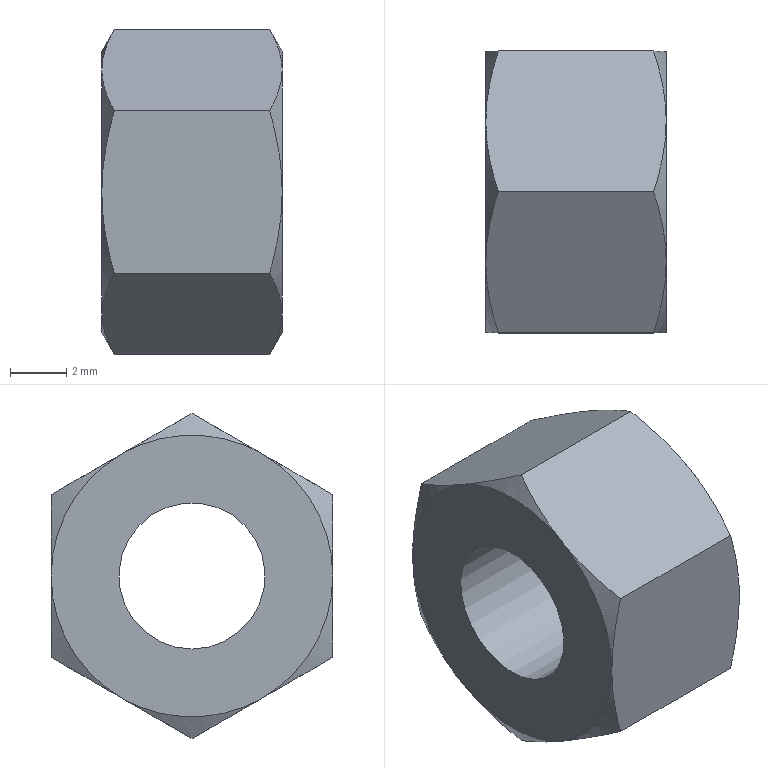Component | NX | GB-T41-2000_M6X1 | 1 solid | 21 faces | volume 417 mm3 | cone 12 | plane 8 | cylinder 1 | commonest cylinder face diameters 5.188 x1